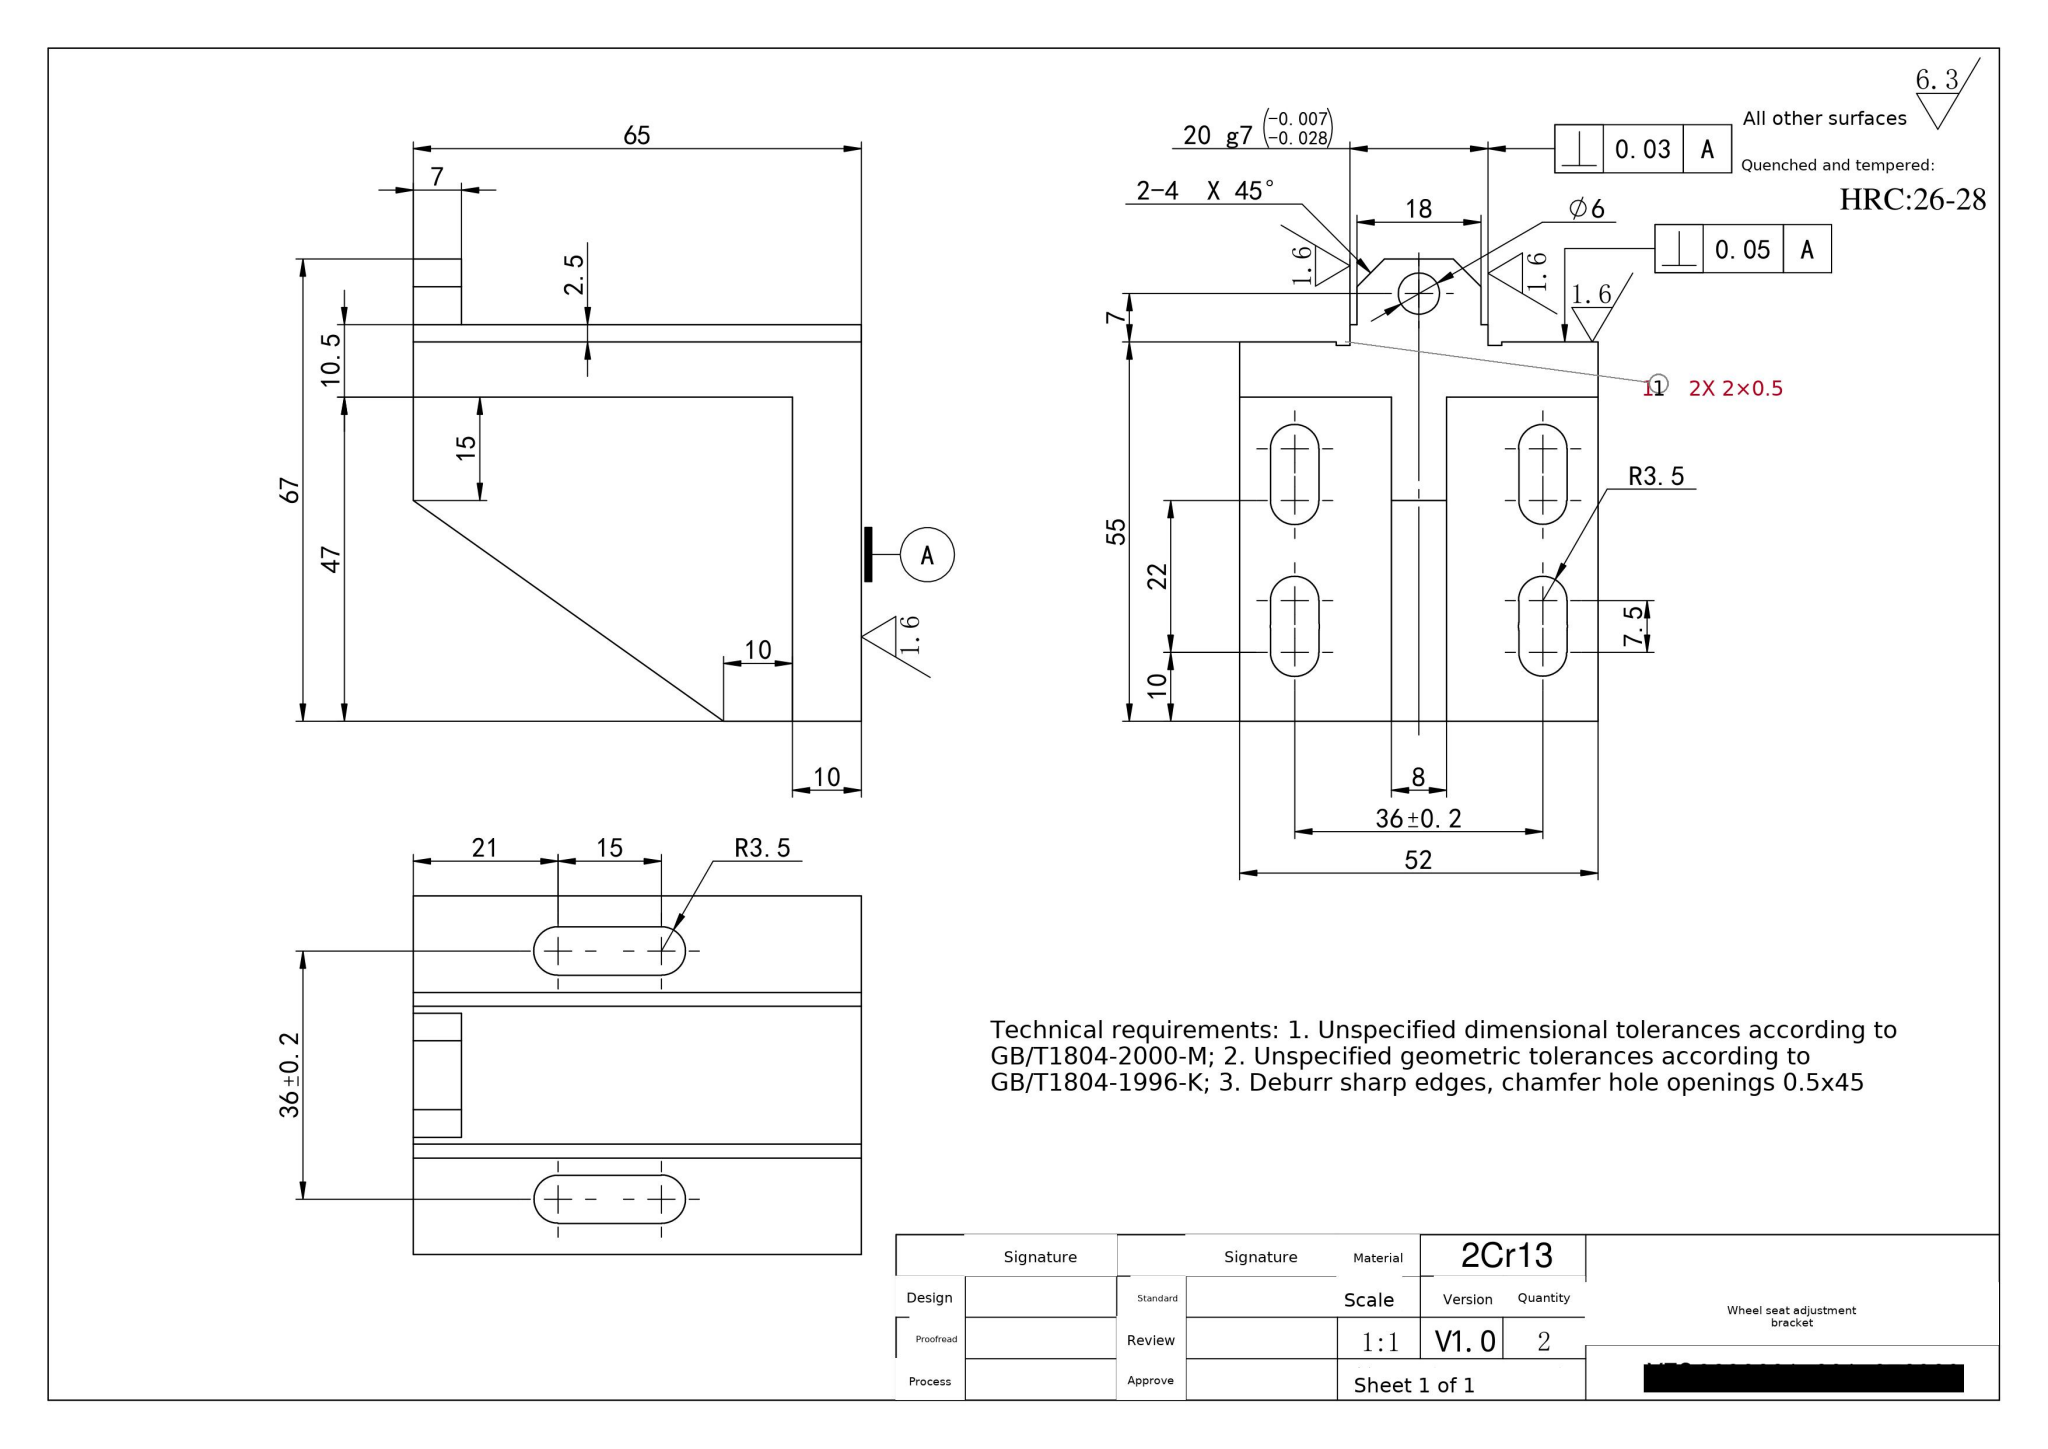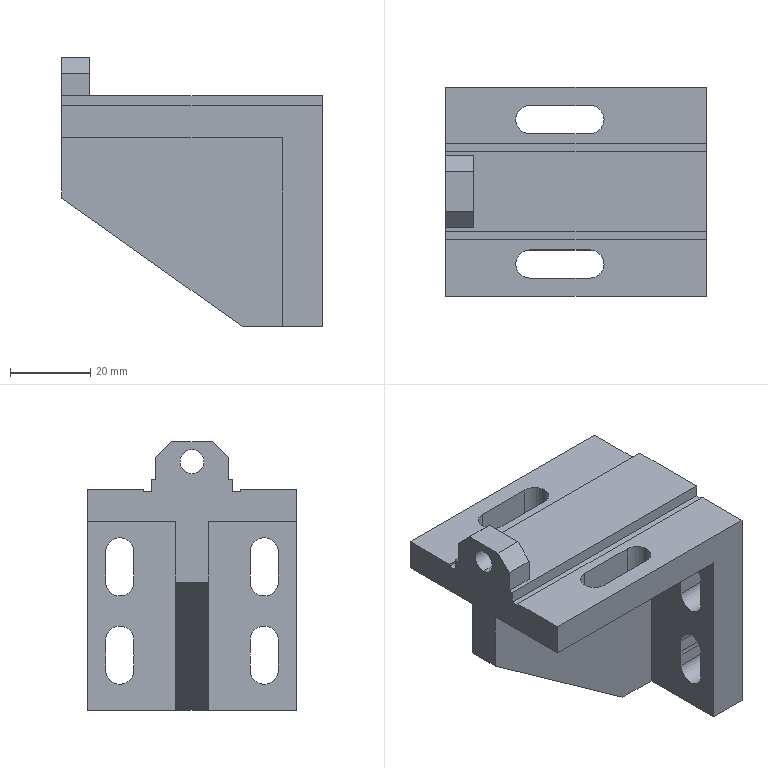Part | SolidWorks | mm | material 2Cr13 | 1 solid | 65 faces | box 65 x 52 x 67 mm | volume 64470 mm3 | plane 43 | cylinder 22 | commonest cylinder face diameters 7 x14 7.1 x6 6 x2